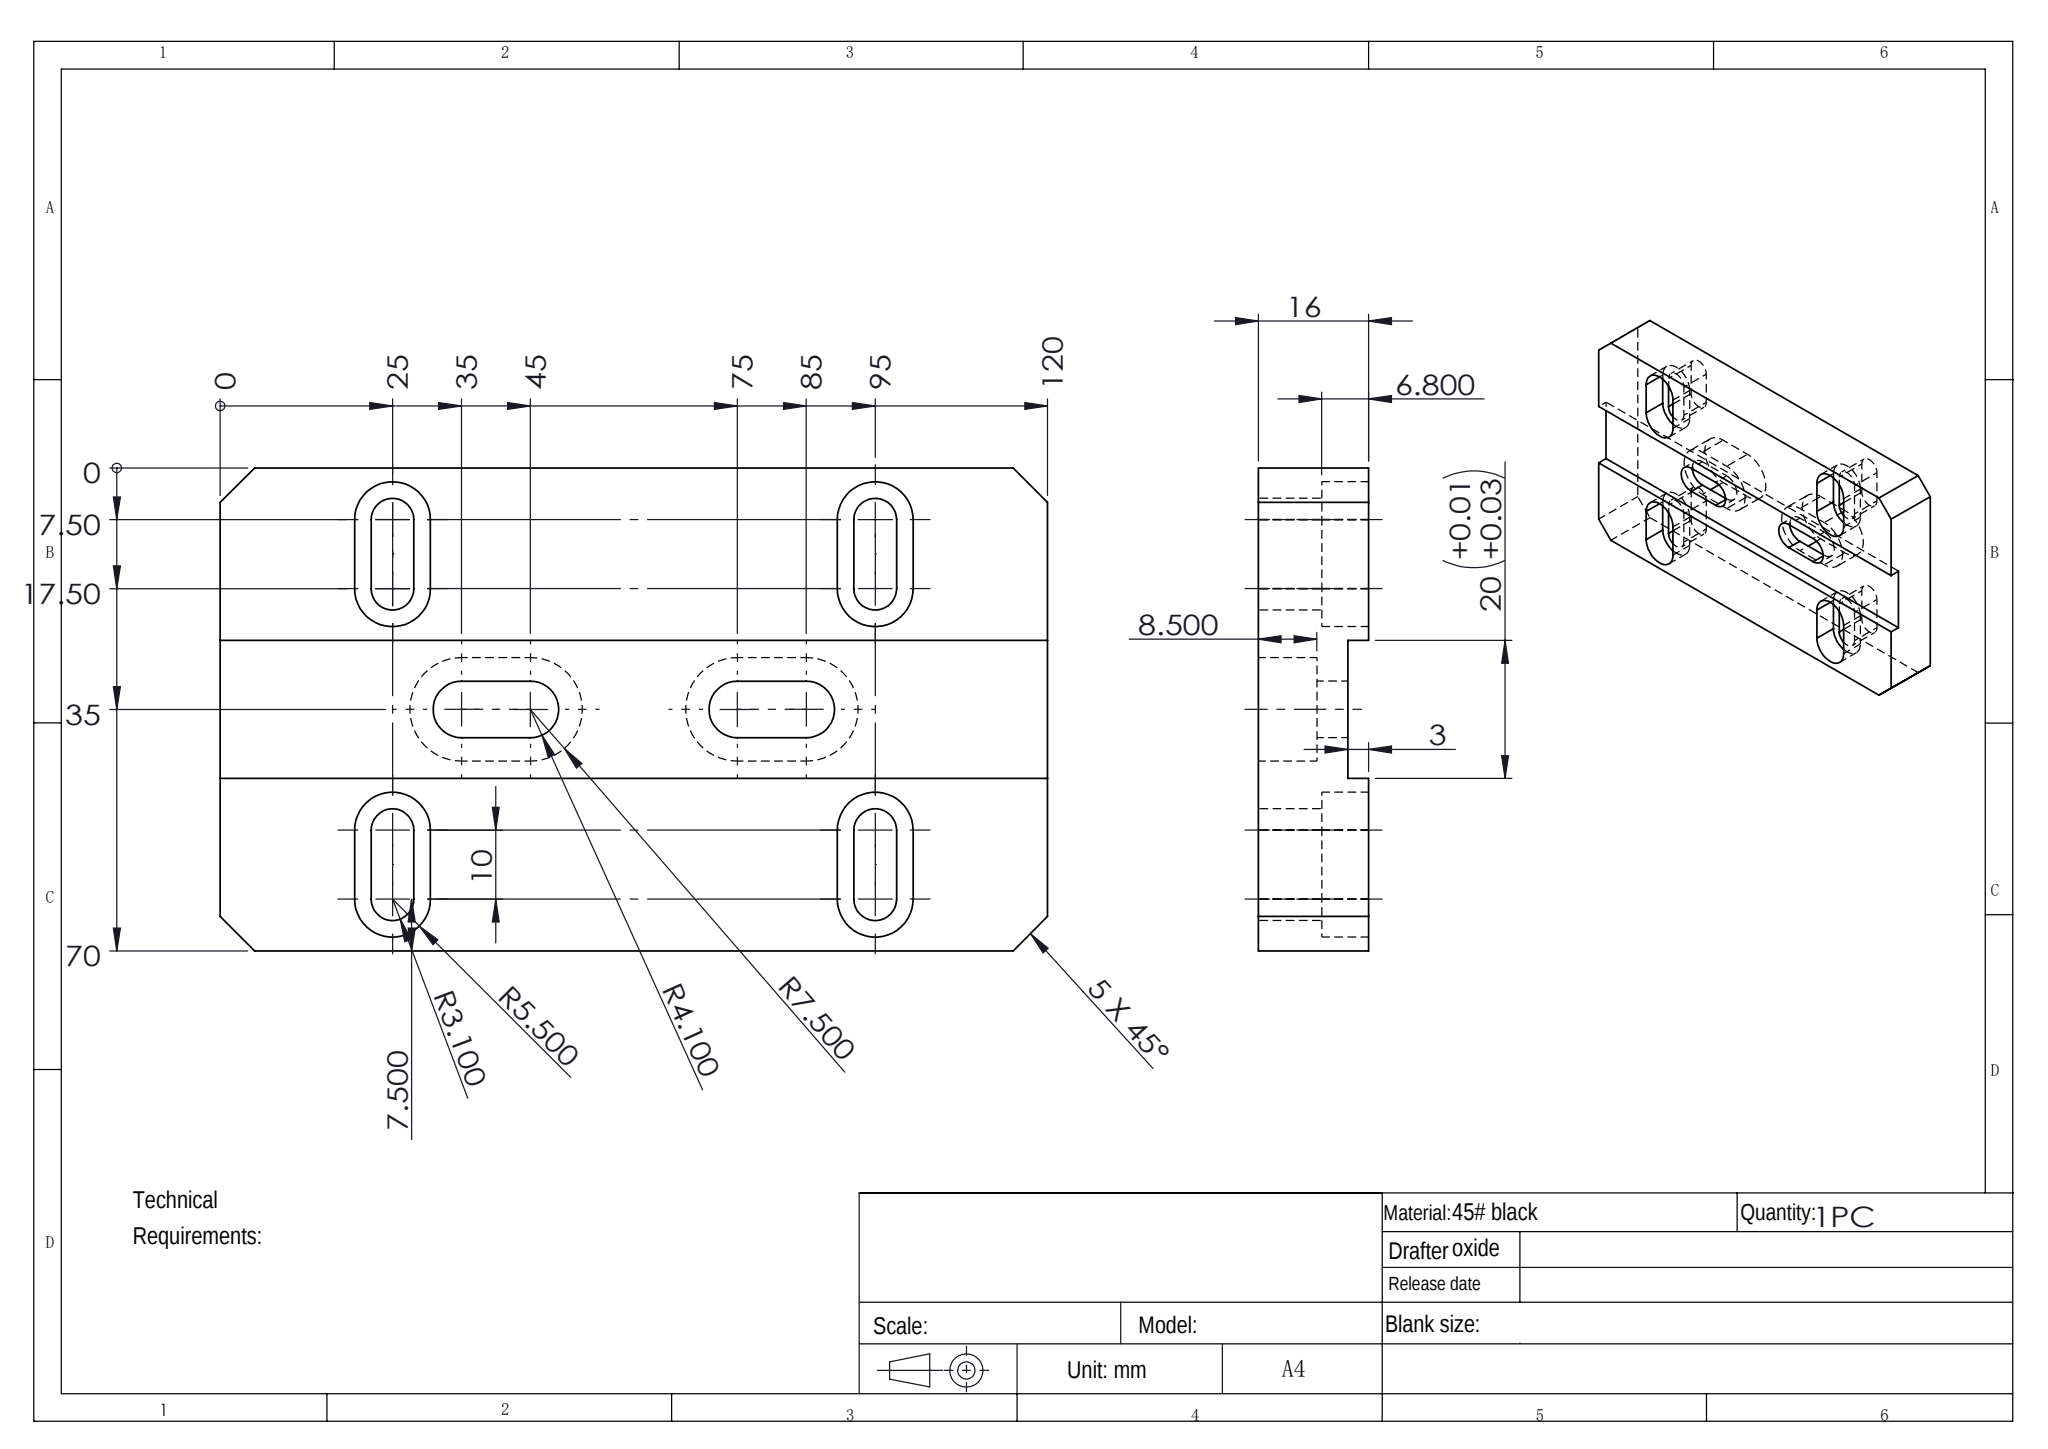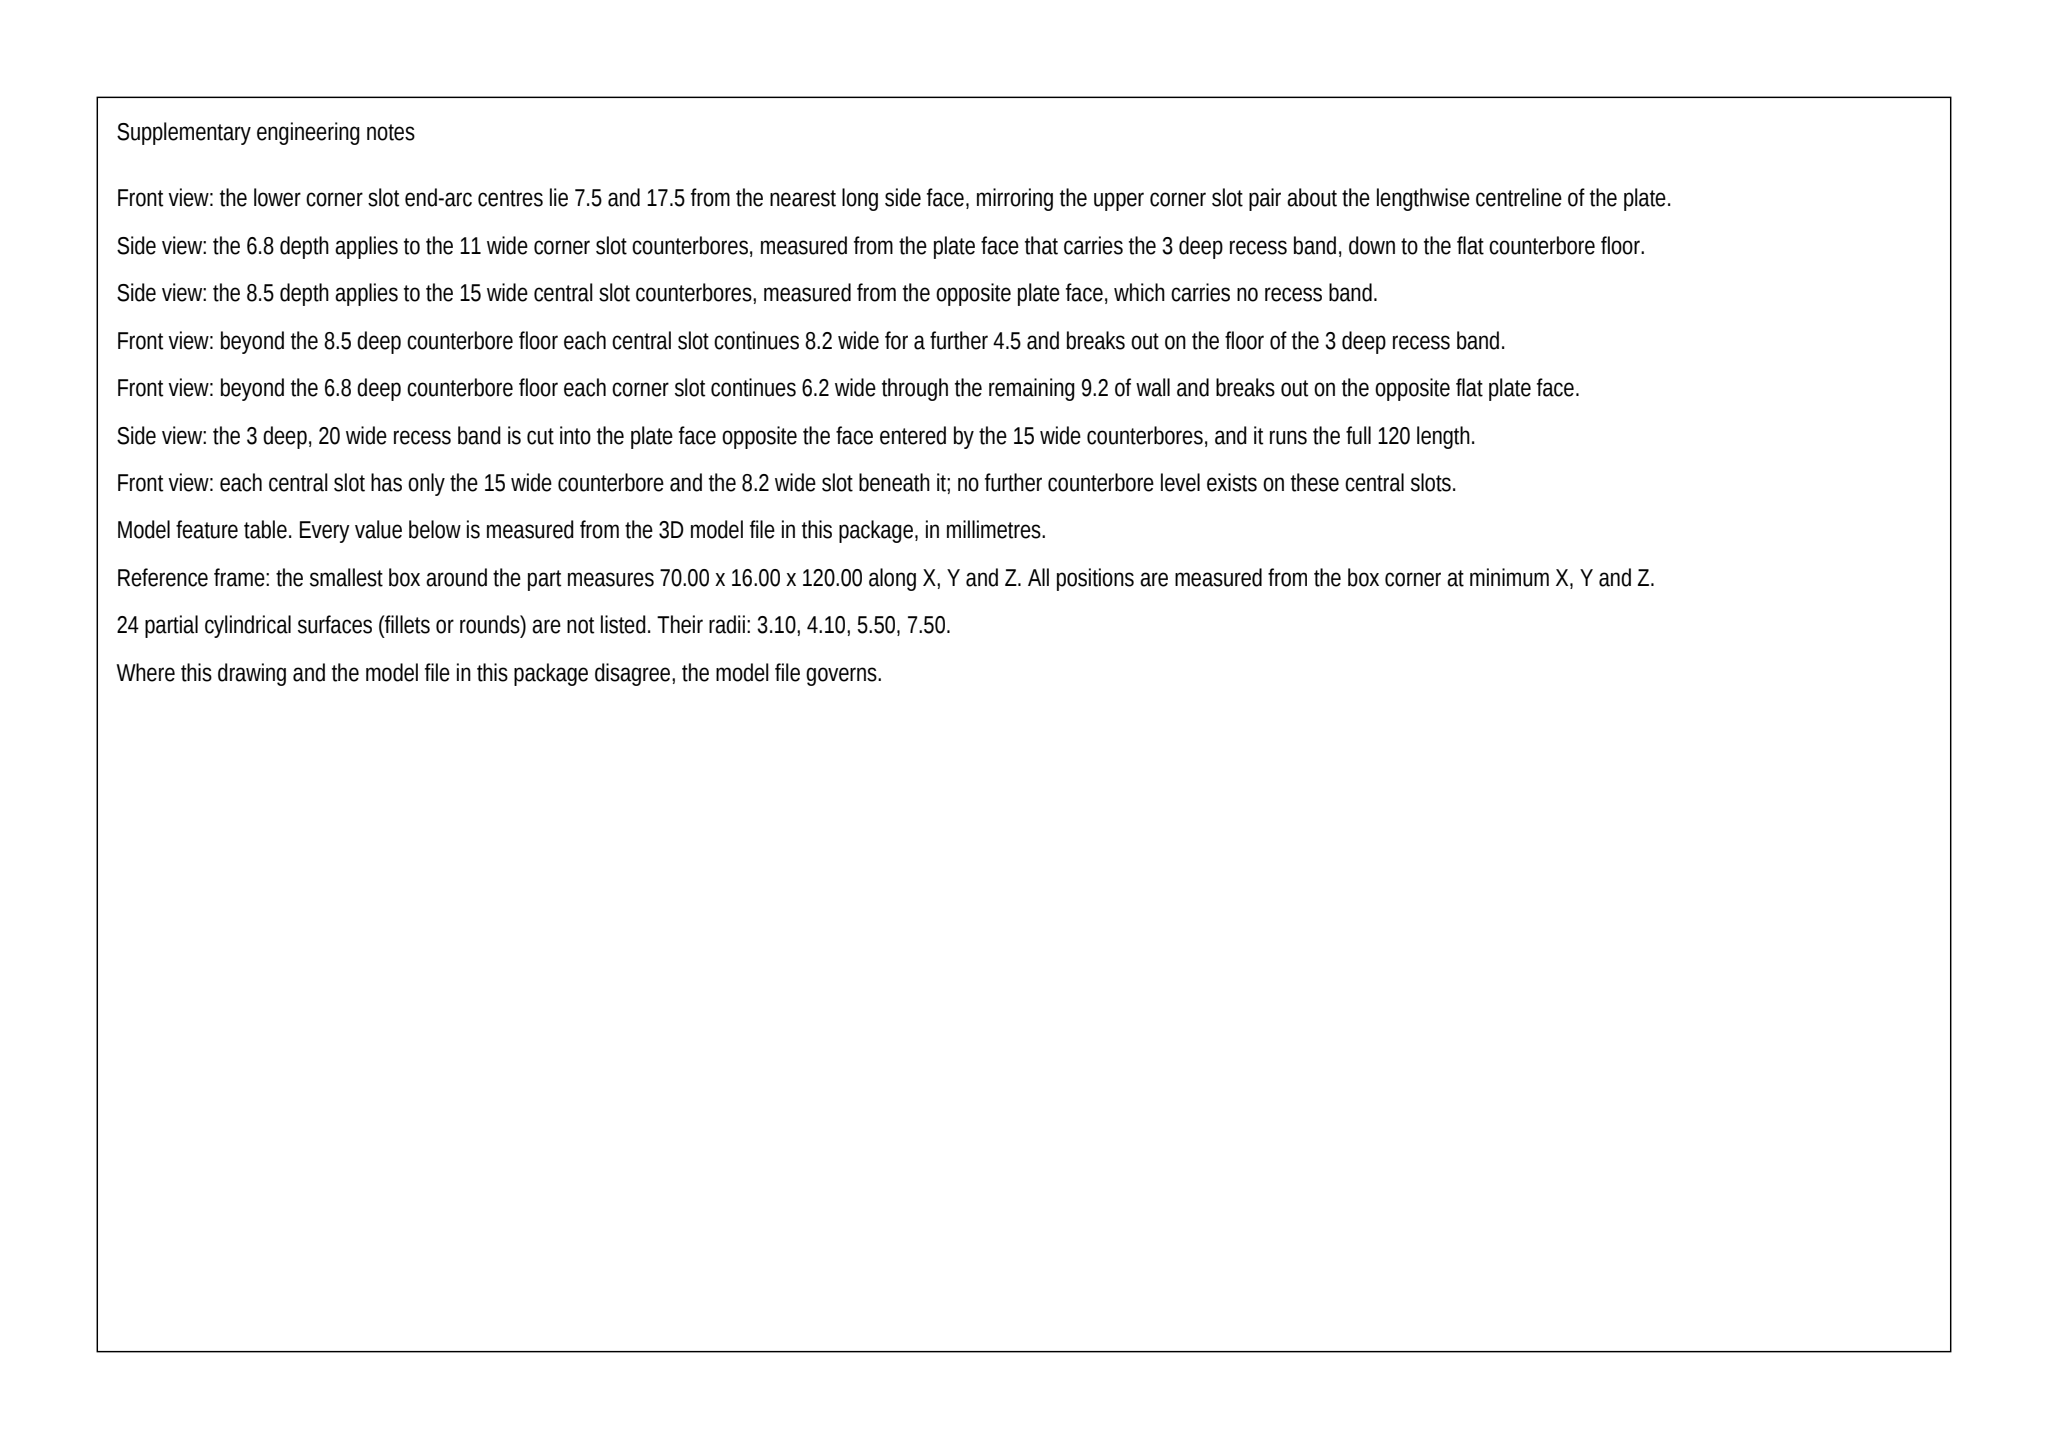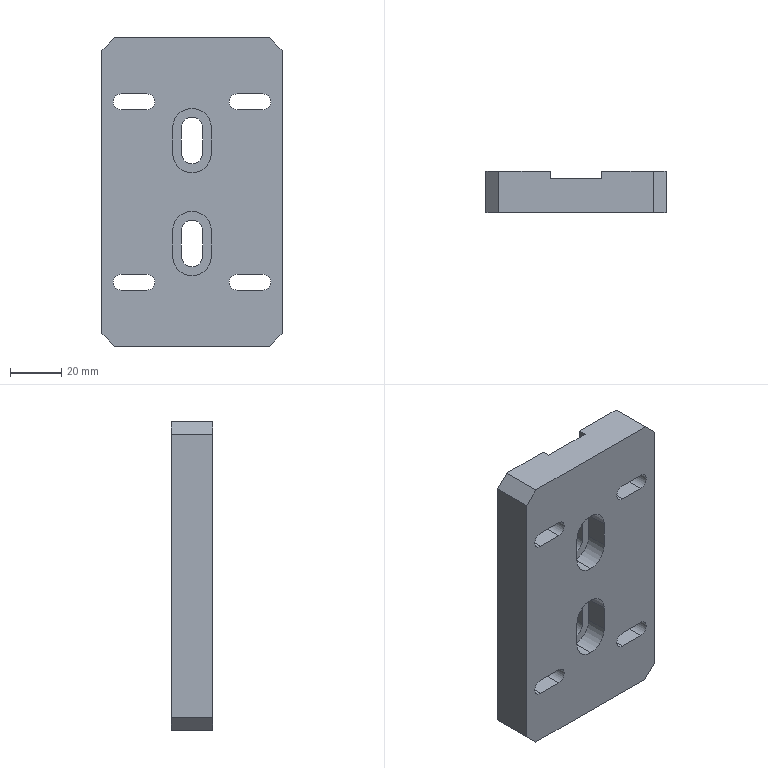Part | SolidWorks | mm | material 45# Blackened | 1 solid | 72 faces | box 70 x 16 x 120 mm | volume 110663 mm3 | plane 44 | cylinder 28 | commonest cylinder face diameters 11 x8 6.2 x8 8.2 x6 15 x6
Drawing notes:
25 FROM TOP EDGE TO EDGE OF 3 DEEP RECESS | from the solid: Plane x=25 (y 13-16, z 0-120) bounds 3 mm deep recess x=25-45; bbox x 0-70
52.50 FROM TOP EDGE TO 1ST END C/L, LWR SLOTS | from the solid: Slot end arcs O11/O6.2 axis y at x=52.5, z=25 & z=95; top edge x=0
62.50 FROM TOP EDGE TO 2ND END C/L, LWR SLOTS | from the solid: Slot end arcs O11/O6.2 axis y at x=62.5, z=25 & z=95; top edge x=0
SLOT END C/L 7.50 FROM NEAREST LONG EDGE, TYP 4 PL | from the solid: End arc centers at x=7.5 and x=62.5 with bbox x 0-70 (70-62.5=7.5)
build123d program:
from build123d import *

# Parameters (mm, degrees)
SKETCH1_W                                            = 70
SKETCH1_H                                            = 16
BOSS_EXTRUDE1_DEPTH                                  = 120
SKETCH2_W                                            = 20
SKETCH2_H                                            = 120
CUT_EXTRUDE1_DEPTH                                   = 3
HOLE_SIZE_ACCORDING_TO_THE_TYPE_OF_HEXAG_D           = 8.2
HOLE_SIZE_ACCORDING_TO_THE_TYPE_OF_HEXAG_CBORE_D     = 15
HOLE_SIZE_ACCORDING_TO_THE_TYPE_OF_HEXAG_CBORE_DEPTH = 8.5
CUT_EXTRUDE2_DEPTH                                   = 8.5
CUT_EXTRUDE3_DEPTH                                   = 82
CHAMFER1_SIZE                                        = 5
HOLE_SIZE_ACCORDING_TO_THE_TYPE_OF_H_2_D             = 6.2
HOLE_SIZE_ACCORDING_TO_THE_TYPE_OF_H_2_CBORE_D       = 11
HOLE_SIZE_ACCORDING_TO_THE_TYPE_OF_H_2_CBORE_DEPTH   = 6.8
CUT_EXTRUDE4_DEPTH                                   = 6.8
CUT_EXTRUDE5_DEPTH                                   = 82
LPATTERN1_COUNT                                      = 2
LPATTERN1_PITCH                                      = 70
LPATTERN1_COUNT_DIR2                                 = 2
LPATTERN1_PITCH_DIR2                                 = 45


with BuildPart() as part:
    # Sketch1 → Boss-Extrude1 (new body)
    with BuildSketch(Plane.XY):
        with Locations((35, 8)):
            Rectangle(SKETCH1_W, SKETCH1_H)
    extrude(amount=BOSS_EXTRUDE1_DEPTH)

    # Sketch2 → Cut-Extrude1 (cut)
    with BuildSketch(Plane(origin=(0, 16, 0), x_dir=(1, 0, 0), z_dir=(0, 1, 0))):
        with Locations((35, -60)):
            Rectangle(SKETCH2_W, SKETCH2_H)
    extrude(amount=-CUT_EXTRUDE1_DEPTH, mode=Mode.SUBTRACT)

    # Hole Size according to the type of hexag (through all)
    with Locations(Plane(origin=(0, 0, 0), x_dir=(-1, 0, 0), z_dir=(0, -1, 0))):
        with Locations((-35, -80), (-35, -40)):
            CounterBoreHole(HOLE_SIZE_ACCORDING_TO_THE_TYPE_OF_HEXAG_D / 2, HOLE_SIZE_ACCORDING_TO_THE_TYPE_OF_HEXAG_CBORE_D / 2, HOLE_SIZE_ACCORDING_TO_THE_TYPE_OF_HEXAG_CBORE_DEPTH)

    # Sketch5 → Cut-Extrude2 (cut)
    with BuildSketch(Plane.XZ):
        with BuildLine():
            Line((27.5, 35), (27.5, 45))
            ThreePointArc((27.5, 45), (35, 52.5), (42.5, 45))
            Line((42.5, 45), (42.5, 35))
            ThreePointArc((42.5, 35), (35, 27.5), (27.5, 35))
        make_face()
        with BuildLine():
            Line((42.5, 85), (42.5, 75))
            ThreePointArc((42.5, 75), (35, 67.5), (27.5, 75))
            Line((27.5, 75), (27.5, 85))
            ThreePointArc((27.5, 85), (35, 92.5), (42.5, 85))
        make_face()
    extrude(amount=-CUT_EXTRUDE2_DEPTH, mode=Mode.SUBTRACT)

    # Sketch6 → Cut-Extrude3 (cut)
    with BuildSketch(Plane.XZ.offset(-8.5)):
        with BuildLine():
            Line((30.9, 75), (30.9, 85))
            ThreePointArc((30.9, 85), (35, 89.1), (39.1, 85))
            Line((39.1, 85), (39.1, 75))
            ThreePointArc((39.1, 75), (35, 70.9), (30.9, 75))
        make_face()
        with BuildLine():
            Line((30.9, 35), (30.9, 45))
            ThreePointArc((30.9, 45), (35, 49.1), (39.1, 45))
            Line((39.1, 45), (39.1, 35))
            ThreePointArc((39.1, 35), (35, 30.9), (30.9, 35))
        make_face()
    extrude(amount=-CUT_EXTRUDE3_DEPTH, mode=Mode.SUBTRACT)

    # Chamfer1
    chamfer1_edges = [part.edges().sort_by_distance(p)[0] for p in [
        (70, 8, 120),
        (0, 8, 120),
        (70, 8, 0),
        (0, 8, 0),
    ]]
    chamfer(chamfer1_edges, length=CHAMFER1_SIZE)

    # Hole Size according to the type of h 2 (through all)
    with Locations(Plane(origin=(0, 16, 0), x_dir=(1, 0, 0), z_dir=(0, 1, 0))):
        with Locations((57.5, -25), (12.5, -25), (12.5, -95), (57.5, -95)):
            CounterBoreHole(HOLE_SIZE_ACCORDING_TO_THE_TYPE_OF_H_2_D / 2, HOLE_SIZE_ACCORDING_TO_THE_TYPE_OF_H_2_CBORE_D / 2, HOLE_SIZE_ACCORDING_TO_THE_TYPE_OF_H_2_CBORE_DEPTH)

    # Sketch9 → Cut-Extrude4 (cut)
    with BuildSketch(Plane(origin=(0, 16, 0), x_dir=(1, 0, 0), z_dir=(0, 1, 0))):
        with BuildLine():
            Line((7.5, -89.5), (17.5, -89.5))
            ThreePointArc((17.5, -89.5), (23, -95), (17.5, -100.5))
            Line((17.5, -100.5), (7.5, -100.5))
            ThreePointArc((7.5, -100.5), (2, -95), (7.5, -89.5))
        make_face()
    cut_extrude4 = extrude(amount=-CUT_EXTRUDE4_DEPTH, mode=Mode.SUBTRACT)

    # Sketch10 → Cut-Extrude5 (cut)
    with BuildSketch(Plane(origin=(0, 9.2, 0), x_dir=(1, 0, 0), z_dir=(0, 1, 0))):
        with BuildLine():
            Line((7.5, -91.9), (17.5, -91.9))
            ThreePointArc((17.5, -91.9), (20.6, -95), (17.5, -98.1))
            Line((17.5, -98.1), (7.5, -98.1))
            ThreePointArc((7.5, -98.1), (4.4, -95), (7.5, -91.9))
        make_face()
    cut_extrude5 = extrude(amount=-CUT_EXTRUDE5_DEPTH, mode=Mode.SUBTRACT)

    # LPattern1: Cut-Extrude4, Cut-Extrude5 2 × 2
    with Locations(*[(j * LPATTERN1_PITCH_DIR2, 0, -i * LPATTERN1_PITCH) for i in range(LPATTERN1_COUNT) for j in range(LPATTERN1_COUNT_DIR2) if (i, j) != (0, 0)]):
        add(cut_extrude4, mode=Mode.SUBTRACT)
        add(cut_extrude5, mode=Mode.SUBTRACT)


solid = part.part